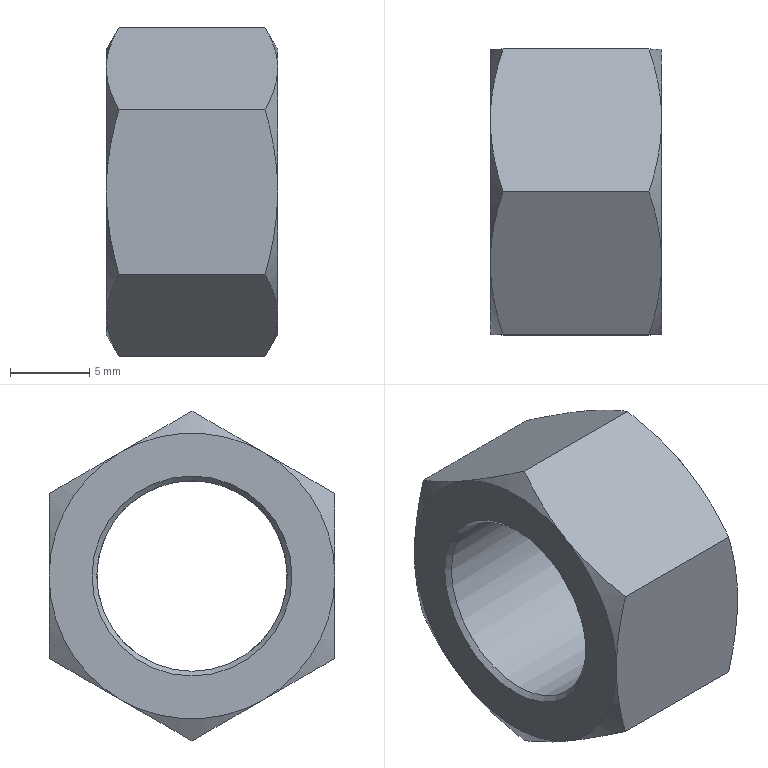Component | NX | GB-T6170_F-2000_M12X1_75_4 | 1 solid | 23 faces | volume 1793 mm3 | cone 14 | plane 8 | cylinder 1 | commonest cylinder face diameters 12 x1